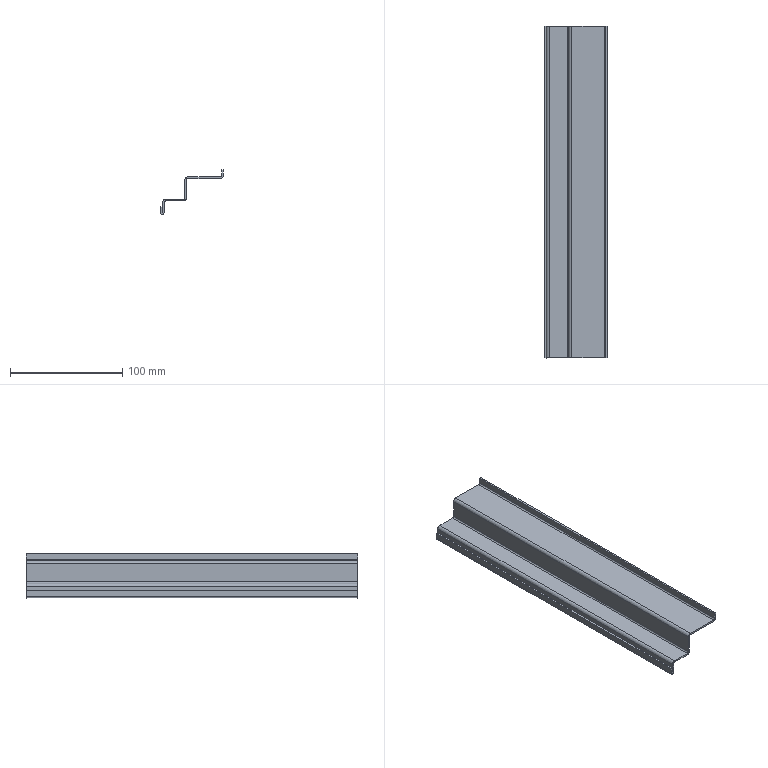Component | SolidWorks | SmallDoorFrameOne100-1 | 1 solid | 46 faces | box 56.1 x 296 x 40 mm | volume 42653 mm3 | plane 36 | cylinder 10 | commonest cylinder face diameters 5.4 x4 2.4 x4 3.1 x1 0.1 x1
STEP:
#1=COLOUR_RGB('',0.7922,0.8196,0.9333);
#2=FILL_AREA_STYLE_COLOUR('',#1);
#3=FILL_AREA_STYLE('',(#2));
#4=SURFACE_STYLE_FILL_AREA(#3);
#5=SURFACE_SIDE_STYLE('',(#4));
#6=SURFACE_STYLE_USAGE(.BOTH.,#5);
#7=PRESENTATION_STYLE_ASSIGNMENT((#6));
#8=CARTESIAN_POINT('',(32.916,29.173,17.246));
#9=VERTEX_POINT('',#8);
#10=CARTESIAN_POINT('',(32.916,29.173,17.61));
#11=VERTEX_POINT('',#10);
#12=CARTESIAN_POINT('',(32.916,29.173,17.185));
#13=DIRECTION('',(-0.,0.,1.));
#14=VECTOR('',#13,39.37);
#15=LINE('',#12,#14);
#16=EDGE_CURVE('',#9,#11,#15,.T.);
#17=ORIENTED_EDGE('',*,*,#16,.F.);
#18=CARTESIAN_POINT('',(32.975,29.173,17.246));
#19=VERTEX_POINT('',#18);
#20=CARTESIAN_POINT('',(32.916,29.173,17.246));
#21=DIRECTION('',(1.,-0.,0.));
#22=VECTOR('',#21,39.37);
#23=LINE('',#20,#22);
#24=EDGE_CURVE('',#9,#19,#23,.T.);
#25=ORIENTED_EDGE('',*,*,#24,.T.);
#26=CARTESIAN_POINT('',(32.975,29.173,17.61));
#27=VERTEX_POINT('',#26);
#28=CARTESIAN_POINT('',(32.975,29.173,17.185));
#29=DIRECTION('',(-0.,0.,1.));
#30=VECTOR('',#29,39.37);
#31=LINE('',#28,#30);
#32=EDGE_CURVE('',#19,#27,#31,.T.);
#33=ORIENTED_EDGE('',*,*,#32,.T.);
#34=CARTESIAN_POINT('',(32.975,29.173,17.61));
#35=DIRECTION('',(-1.,0.,-0.));
#36=VECTOR('',#35,39.37);
#37=LINE('',#34,#36);
#38=EDGE_CURVE('',#27,#11,#37,.T.);
#39=ORIENTED_EDGE('',*,*,#38,.T.);
#40=EDGE_LOOP('',(#17,#25,#33,#39));
#41=FACE_OUTER_BOUND('',#40,.T.);
#42=CARTESIAN_POINT('',(33.022,29.173,17.717));
#43=DIRECTION('',(-0.,-1.,0.));
#44=DIRECTION('',(0.,-0.,-1.));
#45=AXIS2_PLACEMENT_3D('',#42,#43,#44);
#46=PLANE('',#45);
#47=ADVANCED_FACE('',(#41),#46,.T.);
#48=CARTESIAN_POINT('',(33.022,40.827,17.657));
#49=VERTEX_POINT('',#48);
#50=CARTESIAN_POINT('',(33.022,40.827,17.717));
#51=VERTEX_POINT('',#50);
#52=CARTESIAN_POINT('',(33.022,40.827,17.657));
#53=DIRECTION('',(-0.,0.,1.));
#54=VECTOR('',#53,39.37);
#55=LINE('',#52,#54);
#56=EDGE_CURVE('',#49,#51,#55,.T.);
#57=ORIENTED_EDGE('',*,*,#56,.F.);
#58=CARTESIAN_POINT('',(32.975,40.827,17.61));
#59=VERTEX_POINT('',#58);
#60=CARTESIAN_POINT('',(33.022,40.827,17.61));
#61=DIRECTION('',(0.,1.,-0.));
#62=DIRECTION('',(0.,0.,-1.));
#63=AXIS2_PLACEMENT_3D('',#60,#61,#62);
#64=CIRCLE('',#63,0.04724);
#65=EDGE_CURVE('',#59,#49,#64,.T.);
#66=ORIENTED_EDGE('',*,*,#65,.F.);
#67=CARTESIAN_POINT('',(32.916,40.827,17.61));
#68=VERTEX_POINT('',#67);
#69=CARTESIAN_POINT('',(32.916,40.827,17.61));
#70=DIRECTION('',(1.,-0.,0.));
#71=VECTOR('',#70,39.37);
#72=LINE('',#69,#71);
#73=EDGE_CURVE('',#68,#59,#72,.T.);
#74=ORIENTED_EDGE('',*,*,#73,.F.);
#75=CARTESIAN_POINT('',(33.022,40.827,17.61));
#76=DIRECTION('',(0.,1.,-0.));
#77=DIRECTION('',(0.,0.,1.));
#78=AXIS2_PLACEMENT_3D('',#75,#76,#77);
#79=CIRCLE('',#78,0.1063);
#80=EDGE_CURVE('',#68,#51,#79,.T.);
#81=ORIENTED_EDGE('',*,*,#80,.T.);
#82=EDGE_LOOP('',(#57,#66,#74,#81));
#83=FACE_OUTER_BOUND('',#82,.T.);
#84=CARTESIAN_POINT('',(33.022,40.827,17.657));
#85=DIRECTION('',(0.,1.,-0.));
#86=DIRECTION('',(-0.,0.,1.));
#87=AXIS2_PLACEMENT_3D('',#84,#85,#86);
#88=PLANE('',#87);
#89=ADVANCED_FACE('',(#83),#88,.T.);
#90=CARTESIAN_POINT('',(33.656,40.827,17.657));
#91=VERTEX_POINT('',#90);
#92=CARTESIAN_POINT('',(32.975,40.827,17.657));
#93=DIRECTION('',(1.,-0.,0.));
#94=VECTOR('',#93,39.37);
#95=LINE('',#92,#94);
#96=EDGE_CURVE('',#49,#91,#95,.T.);
#97=ORIENTED_EDGE('',*,*,#96,.F.);
#98=ORIENTED_EDGE('',*,*,#56,.T.);
#99=CARTESIAN_POINT('',(33.656,40.827,17.717));
#100=VERTEX_POINT('',#99);
#101=CARTESIAN_POINT('',(32.975,40.827,17.717));
#102=DIRECTION('',(1.,-0.,0.));
#103=VECTOR('',#102,39.37);
#104=LINE('',#101,#103);
#105=EDGE_CURVE('',#51,#100,#104,.T.);
#106=ORIENTED_EDGE('',*,*,#105,.T.);
#107=CARTESIAN_POINT('',(33.656,40.827,17.717));
#108=DIRECTION('',(0.,-0.,-1.));
#109=VECTOR('',#108,39.37);
#110=LINE('',#107,#109);
#111=EDGE_CURVE('',#100,#91,#110,.T.);
#112=ORIENTED_EDGE('',*,*,#111,.T.);
#113=EDGE_LOOP('',(#97,#98,#106,#112));
#114=FACE_OUTER_BOUND('',#113,.T.);
#115=CARTESIAN_POINT('',(32.916,40.827,17.61));
#116=DIRECTION('',(0.,1.,-0.));
#117=DIRECTION('',(-0.,0.,1.));
#118=AXIS2_PLACEMENT_3D('',#115,#116,#117);
#119=PLANE('',#118);
#120=ADVANCED_FACE('',(#114),#119,.T.);
#121=ORIENTED_EDGE('',*,*,#38,.F.);
#122=CARTESIAN_POINT('',(33.022,29.173,17.657));
#123=VERTEX_POINT('',#122);
#124=CARTESIAN_POINT('',(33.022,29.173,17.61));
#125=DIRECTION('',(0.,1.,-0.));
#126=DIRECTION('',(0.,0.,-1.));
#127=AXIS2_PLACEMENT_3D('',#124,#125,#126);
#128=CIRCLE('',#127,0.04724);
#129=EDGE_CURVE('',#27,#123,#128,.T.);
#130=ORIENTED_EDGE('',*,*,#129,.T.);
#131=CARTESIAN_POINT('',(33.022,29.173,17.717));
#132=VERTEX_POINT('',#131);
#133=CARTESIAN_POINT('',(33.022,29.173,17.717));
#134=DIRECTION('',(0.,-0.,-1.));
#135=VECTOR('',#134,39.37);
#136=LINE('',#133,#135);
#137=EDGE_CURVE('',#132,#123,#136,.T.);
#138=ORIENTED_EDGE('',*,*,#137,.F.);
#139=CARTESIAN_POINT('',(33.022,29.173,17.61));
#140=DIRECTION('',(0.,1.,-0.));
#141=DIRECTION('',(0.,0.,1.));
#142=AXIS2_PLACEMENT_3D('',#139,#140,#141);
#143=CIRCLE('',#142,0.1063);
#144=EDGE_CURVE('',#11,#132,#143,.T.);
#145=ORIENTED_EDGE('',*,*,#144,.F.);
#146=EDGE_LOOP('',(#121,#130,#138,#145));
#147=FACE_OUTER_BOUND('',#146,.T.);
#148=CARTESIAN_POINT('',(32.975,29.173,17.61));
#149=DIRECTION('',(-0.,-1.,0.));
#150=DIRECTION('',(0.,-0.,-1.));
#151=AXIS2_PLACEMENT_3D('',#148,#149,#150);
#152=PLANE('',#151);
#153=ADVANCED_FACE('',(#147),#152,.T.);
#154=CARTESIAN_POINT('',(33.762,40.827,17.764));
#155=VERTEX_POINT('',#154);
#156=CARTESIAN_POINT('',(33.703,40.827,17.764));
#157=VERTEX_POINT('',#156);
#158=CARTESIAN_POINT('',(33.762,40.827,17.764));
#159=DIRECTION('',(-1.,0.,-0.));
#160=VECTOR('',#159,39.37);
#161=LINE('',#158,#160);
#162=EDGE_CURVE('',#155,#157,#161,.T.);
#163=ORIENTED_EDGE('',*,*,#162,.F.);
#164=CARTESIAN_POINT('',(33.656,40.827,17.764));
#165=DIRECTION('',(-0.,-1.,0.));
#166=DIRECTION('',(0.,0.,1.));
#167=AXIS2_PLACEMENT_3D('',#164,#165,#166);
#168=CIRCLE('',#167,0.1063);
#169=EDGE_CURVE('',#91,#155,#168,.T.);
#170=ORIENTED_EDGE('',*,*,#169,.F.);
#171=ORIENTED_EDGE('',*,*,#111,.F.);
#172=CARTESIAN_POINT('',(33.656,40.827,17.764));
#173=DIRECTION('',(-0.,-1.,0.));
#174=DIRECTION('',(0.,0.,1.));
#175=AXIS2_PLACEMENT_3D('',#172,#173,#174);
#176=CIRCLE('',#175,0.04724);
#177=EDGE_CURVE('',#100,#157,#176,.T.);
#178=ORIENTED_EDGE('',*,*,#177,.T.);
#179=EDGE_LOOP('',(#163,#170,#171,#178));
#180=FACE_OUTER_BOUND('',#179,.T.);
#181=CARTESIAN_POINT('',(33.762,40.827,17.764));
#182=DIRECTION('',(0.,1.,-0.));
#183=DIRECTION('',(-0.,0.,1.));
#184=AXIS2_PLACEMENT_3D('',#181,#182,#183);
#185=PLANE('',#184);
#186=ADVANCED_FACE('',(#180),#185,.T.);
#187=CARTESIAN_POINT('',(33.762,40.827,18.398));
#188=VERTEX_POINT('',#187);
#189=CARTESIAN_POINT('',(33.762,40.827,17.657));
#190=DIRECTION('',(-0.,0.,1.));
#191=VECTOR('',#190,39.37);
#192=LINE('',#189,#191);
#193=EDGE_CURVE('',#155,#188,#192,.T.);
#194=ORIENTED_EDGE('',*,*,#193,.F.);
#195=ORIENTED_EDGE('',*,*,#162,.T.);
#196=CARTESIAN_POINT('',(33.703,40.827,18.398));
#197=VERTEX_POINT('',#196);
#198=CARTESIAN_POINT('',(33.703,40.827,17.657));
#199=DIRECTION('',(-0.,0.,1.));
#200=VECTOR('',#199,39.37);
#201=LINE('',#198,#200);
#202=EDGE_CURVE('',#157,#197,#201,.T.);
#203=ORIENTED_EDGE('',*,*,#202,.T.);
#204=CARTESIAN_POINT('',(33.703,40.827,18.398));
#205=DIRECTION('',(1.,-0.,0.));
#206=VECTOR('',#205,39.37);
#207=LINE('',#204,#206);
#208=EDGE_CURVE('',#197,#188,#207,.T.);
#209=ORIENTED_EDGE('',*,*,#208,.T.);
#210=EDGE_LOOP('',(#194,#195,#203,#209));
#211=FACE_OUTER_BOUND('',#210,.T.);
#212=CARTESIAN_POINT('',(33.656,40.827,17.717));
#213=DIRECTION('',(0.,1.,-0.));
#214=DIRECTION('',(-0.,0.,1.));
#215=AXIS2_PLACEMENT_3D('',#212,#213,#214);
#216=PLANE('',#215);
#217=ADVANCED_FACE('',(#211),#216,.T.);
#218=CARTESIAN_POINT('',(33.656,29.173,17.657));
#219=VERTEX_POINT('',#218);
#220=CARTESIAN_POINT('',(33.656,29.173,17.717));
#221=VERTEX_POINT('',#220);
#222=CARTESIAN_POINT('',(33.656,29.173,17.657));
#223=DIRECTION('',(-0.,0.,1.));
#224=VECTOR('',#223,39.37);
#225=LINE('',#222,#224);
#226=EDGE_CURVE('',#219,#221,#225,.T.);
#227=ORIENTED_EDGE('',*,*,#226,.F.);
#228=CARTESIAN_POINT('',(33.762,29.173,17.764));
#229=VERTEX_POINT('',#228);
#230=CARTESIAN_POINT('',(33.656,29.173,17.764));
#231=DIRECTION('',(-0.,-1.,0.));
#232=DIRECTION('',(0.,0.,1.));
#233=AXIS2_PLACEMENT_3D('',#230,#231,#232);
#234=CIRCLE('',#233,0.1063);
#235=EDGE_CURVE('',#219,#229,#234,.T.);
#236=ORIENTED_EDGE('',*,*,#235,.T.);
#237=CARTESIAN_POINT('',(33.703,29.173,17.764));
#238=VERTEX_POINT('',#237);
#239=CARTESIAN_POINT('',(33.703,29.173,17.764));
#240=DIRECTION('',(1.,-0.,0.));
#241=VECTOR('',#240,39.37);
#242=LINE('',#239,#241);
#243=EDGE_CURVE('',#238,#229,#242,.T.);
#244=ORIENTED_EDGE('',*,*,#243,.F.);
#245=CARTESIAN_POINT('',(33.656,29.173,17.764));
#246=DIRECTION('',(-0.,-1.,0.));
#247=DIRECTION('',(0.,0.,1.));
#248=AXIS2_PLACEMENT_3D('',#245,#246,#247);
#249=CIRCLE('',#248,0.04724);
#250=EDGE_CURVE('',#221,#238,#249,.T.);
#251=ORIENTED_EDGE('',*,*,#250,.F.);
#252=EDGE_LOOP('',(#227,#236,#244,#251));
#253=FACE_OUTER_BOUND('',#252,.T.);
#254=CARTESIAN_POINT('',(33.656,29.173,17.657));
#255=DIRECTION('',(-0.,-1.,0.));
#256=DIRECTION('',(0.,-0.,-1.));
#257=AXIS2_PLACEMENT_3D('',#254,#255,#256);
#258=PLANE('',#257);
#259=ADVANCED_FACE('',(#253),#258,.T.);
#260=CARTESIAN_POINT('',(32.975,29.173,17.657));
#261=DIRECTION('',(1.,-0.,0.));
#262=VECTOR('',#261,39.37);
#263=LINE('',#260,#262);
#264=EDGE_CURVE('',#123,#219,#263,.T.);
#265=ORIENTED_EDGE('',*,*,#264,.T.);
#266=ORIENTED_EDGE('',*,*,#226,.T.);
#267=CARTESIAN_POINT('',(32.975,29.173,17.717));
#268=DIRECTION('',(1.,-0.,0.));
#269=VECTOR('',#268,39.37);
#270=LINE('',#267,#269);
#271=EDGE_CURVE('',#132,#221,#270,.T.);
#272=ORIENTED_EDGE('',*,*,#271,.F.);
#273=ORIENTED_EDGE('',*,*,#137,.T.);
#274=EDGE_LOOP('',(#265,#266,#272,#273));
#275=FACE_OUTER_BOUND('',#274,.T.);
#276=CARTESIAN_POINT('',(33.703,29.173,17.764));
#277=DIRECTION('',(-0.,-1.,0.));
#278=DIRECTION('',(0.,-0.,-1.));
#279=AXIS2_PLACEMENT_3D('',#276,#277,#278);
#280=PLANE('',#279);
#281=ADVANCED_FACE('',(#275),#280,.T.);
#282=CARTESIAN_POINT('',(33.809,40.827,18.445));
#283=VERTEX_POINT('',#282);
#284=CARTESIAN_POINT('',(33.809,40.827,18.504));
#285=VERTEX_POINT('',#284);
#286=CARTESIAN_POINT('',(33.809,40.827,18.445));
#287=DIRECTION('',(-0.,0.,1.));
#288=VECTOR('',#287,39.37);
#289=LINE('',#286,#288);
#290=EDGE_CURVE('',#283,#285,#289,.T.);
#291=ORIENTED_EDGE('',*,*,#290,.F.);
#292=CARTESIAN_POINT('',(33.809,40.827,18.398));
#293=DIRECTION('',(0.,1.,-0.));
#294=DIRECTION('',(0.,0.,-1.));
#295=AXIS2_PLACEMENT_3D('',#292,#293,#294);
#296=CIRCLE('',#295,0.04724);
#297=EDGE_CURVE('',#188,#283,#296,.T.);
#298=ORIENTED_EDGE('',*,*,#297,.F.);
#299=ORIENTED_EDGE('',*,*,#208,.F.);
#300=CARTESIAN_POINT('',(33.809,40.827,18.398));
#301=DIRECTION('',(0.,1.,-0.));
#302=DIRECTION('',(0.,0.,1.));
#303=AXIS2_PLACEMENT_3D('',#300,#301,#302);
#304=CIRCLE('',#303,0.1063);
#305=EDGE_CURVE('',#197,#285,#304,.T.);
#306=ORIENTED_EDGE('',*,*,#305,.T.);
#307=EDGE_LOOP('',(#291,#298,#299,#306));
#308=FACE_OUTER_BOUND('',#307,.T.);
#309=CARTESIAN_POINT('',(33.809,40.827,18.445));
#310=DIRECTION('',(0.,1.,-0.));
#311=DIRECTION('',(-0.,0.,1.));
#312=AXIS2_PLACEMENT_3D('',#309,#310,#311);
#313=PLANE('',#312);
#314=ADVANCED_FACE('',(#308),#313,.T.);
#315=CARTESIAN_POINT('',(34.955,40.827,18.445));
#316=VERTEX_POINT('',#315);
#317=CARTESIAN_POINT('',(33.762,40.827,18.445));
#318=DIRECTION('',(1.,-0.,0.));
#319=VECTOR('',#318,39.37);
#320=LINE('',#317,#319);
#321=EDGE_CURVE('',#283,#316,#320,.T.);
#322=ORIENTED_EDGE('',*,*,#321,.F.);
#323=ORIENTED_EDGE('',*,*,#290,.T.);
#324=CARTESIAN_POINT('',(34.955,40.827,18.504));
#325=VERTEX_POINT('',#324);
#326=CARTESIAN_POINT('',(33.762,40.827,18.504));
#327=DIRECTION('',(1.,-0.,0.));
#328=VECTOR('',#327,39.37);
#329=LINE('',#326,#328);
#330=EDGE_CURVE('',#285,#325,#329,.T.);
#331=ORIENTED_EDGE('',*,*,#330,.T.);
#332=CARTESIAN_POINT('',(34.955,40.827,18.504));
#333=DIRECTION('',(0.,-0.,-1.));
#334=VECTOR('',#333,39.37);
#335=LINE('',#332,#334);
#336=EDGE_CURVE('',#325,#316,#335,.T.);
#337=ORIENTED_EDGE('',*,*,#336,.T.);
#338=EDGE_LOOP('',(#322,#323,#331,#337));
#339=FACE_OUTER_BOUND('',#338,.T.);
#340=CARTESIAN_POINT('',(33.703,40.827,18.398));
#341=DIRECTION('',(0.,1.,-0.));
#342=DIRECTION('',(-0.,0.,1.));
#343=AXIS2_PLACEMENT_3D('',#340,#341,#342);
#344=PLANE('',#343);
#345=ADVANCED_FACE('',(#339),#344,.T.);
#346=CARTESIAN_POINT('',(33.762,29.173,18.398));
#347=VERTEX_POINT('',#346);
#348=CARTESIAN_POINT('',(33.703,29.173,18.398));
#349=VERTEX_POINT('',#348);
#350=CARTESIAN_POINT('',(33.762,29.173,18.398));
#351=DIRECTION('',(-1.,0.,-0.));
#352=VECTOR('',#351,39.37);
#353=LINE('',#350,#352);
#354=EDGE_CURVE('',#347,#349,#353,.T.);
#355=ORIENTED_EDGE('',*,*,#354,.F.);
#356=CARTESIAN_POINT('',(33.809,29.173,18.445));
#357=VERTEX_POINT('',#356);
#358=CARTESIAN_POINT('',(33.809,29.173,18.398));
#359=DIRECTION('',(0.,1.,-0.));
#360=DIRECTION('',(0.,0.,-1.));
#361=AXIS2_PLACEMENT_3D('',#358,#359,#360);
#362=CIRCLE('',#361,0.04724);
#363=EDGE_CURVE('',#347,#357,#362,.T.);
#364=ORIENTED_EDGE('',*,*,#363,.T.);
#365=CARTESIAN_POINT('',(33.809,29.173,18.504));
#366=VERTEX_POINT('',#365);
#367=CARTESIAN_POINT('',(33.809,29.173,18.504));
#368=DIRECTION('',(0.,-0.,-1.));
#369=VECTOR('',#368,39.37);
#370=LINE('',#367,#369);
#371=EDGE_CURVE('',#366,#357,#370,.T.);
#372=ORIENTED_EDGE('',*,*,#371,.F.);
#373=CARTESIAN_POINT('',(33.809,29.173,18.398));
#374=DIRECTION('',(0.,1.,-0.));
#375=DIRECTION('',(0.,0.,1.));
#376=AXIS2_PLACEMENT_3D('',#373,#374,#375);
#377=CIRCLE('',#376,0.1063);
#378=EDGE_CURVE('',#349,#366,#377,.T.);
#379=ORIENTED_EDGE('',*,*,#378,.F.);
#380=EDGE_LOOP('',(#355,#364,#372,#379));
#381=FACE_OUTER_BOUND('',#380,.T.);
#382=CARTESIAN_POINT('',(33.762,29.173,18.398));
#383=DIRECTION('',(-0.,-1.,0.));
#384=DIRECTION('',(0.,-0.,-1.));
#385=AXIS2_PLACEMENT_3D('',#382,#383,#384);
#386=PLANE('',#385);
#387=ADVANCED_FACE('',(#381),#386,.T.);
#388=CARTESIAN_POINT('',(33.762,29.173,17.657));
#389=DIRECTION('',(-0.,0.,1.));
#390=VECTOR('',#389,39.37);
#391=LINE('',#388,#390);
#392=EDGE_CURVE('',#229,#347,#391,.T.);
#393=ORIENTED_EDGE('',*,*,#392,.T.);
#394=ORIENTED_EDGE('',*,*,#354,.T.);
#395=CARTESIAN_POINT('',(33.703,29.173,17.657));
#396=DIRECTION('',(-0.,0.,1.));
#397=VECTOR('',#396,39.37);
#398=LINE('',#395,#397);
#399=EDGE_CURVE('',#238,#349,#398,.T.);
#400=ORIENTED_EDGE('',*,*,#399,.F.);
#401=ORIENTED_EDGE('',*,*,#243,.T.);
#402=EDGE_LOOP('',(#393,#394,#400,#401));
#403=FACE_OUTER_BOUND('',#402,.T.);
#404=CARTESIAN_POINT('',(33.809,29.173,18.504));
#405=DIRECTION('',(-0.,-1.,0.));
#406=DIRECTION('',(0.,-0.,-1.));
#407=AXIS2_PLACEMENT_3D('',#404,#405,#406);
#408=PLANE('',#407);
#409=ADVANCED_FACE('',(#403),#408,.T.);
#410=CARTESIAN_POINT('',(35.061,40.827,18.551));
#411=VERTEX_POINT('',#410);
#412=CARTESIAN_POINT('',(35.002,40.827,18.551));
#413=VERTEX_POINT('',#412);
#414=CARTESIAN_POINT('',(35.061,40.827,18.551));
#415=DIRECTION('',(-1.,0.,-0.));
#416=VECTOR('',#415,39.37);
#417=LINE('',#414,#416);
#418=EDGE_CURVE('',#411,#413,#417,.T.);
#419=ORIENTED_EDGE('',*,*,#418,.F.);
#420=CARTESIAN_POINT('',(34.955,40.827,18.551));
#421=DIRECTION('',(-0.,-1.,0.));
#422=DIRECTION('',(0.,0.,1.));
#423=AXIS2_PLACEMENT_3D('',#420,#421,#422);
#424=CIRCLE('',#423,0.1063);
#425=EDGE_CURVE('',#316,#411,#424,.T.);
#426=ORIENTED_EDGE('',*,*,#425,.F.);
#427=ORIENTED_EDGE('',*,*,#336,.F.);
#428=CARTESIAN_POINT('',(34.955,40.827,18.551));
#429=DIRECTION('',(-0.,-1.,0.));
#430=DIRECTION('',(0.,0.,1.));
#431=AXIS2_PLACEMENT_3D('',#428,#429,#430);
#432=CIRCLE('',#431,0.04724);
#433=EDGE_CURVE('',#325,#413,#432,.T.);
#434=ORIENTED_EDGE('',*,*,#433,.T.);
#435=EDGE_LOOP('',(#419,#426,#427,#434));
#436=FACE_OUTER_BOUND('',#435,.T.);
#437=CARTESIAN_POINT('',(35.061,40.827,18.551));
#438=DIRECTION('',(0.,1.,-0.));
#439=DIRECTION('',(-0.,0.,1.));
#440=AXIS2_PLACEMENT_3D('',#437,#438,#439);
#441=PLANE('',#440);
#442=ADVANCED_FACE('',(#436),#441,.T.);
#443=CARTESIAN_POINT('',(35.061,40.827,18.76));
#444=VERTEX_POINT('',#443);
#445=CARTESIAN_POINT('',(35.061,40.827,18.445));
#446=DIRECTION('',(-0.,0.,1.));
#447=VECTOR('',#446,39.37);
#448=LINE('',#445,#447);
#449=EDGE_CURVE('',#411,#444,#448,.T.);
#450=ORIENTED_EDGE('',*,*,#449,.F.);
#451=ORIENTED_EDGE('',*,*,#418,.T.);
#452=CARTESIAN_POINT('',(35.002,40.827,18.76));
#453=VERTEX_POINT('',#452);
#454=CARTESIAN_POINT('',(35.002,40.827,18.445));
#455=DIRECTION('',(-0.,0.,1.));
#456=VECTOR('',#455,39.37);
#457=LINE('',#454,#456);
#458=EDGE_CURVE('',#413,#453,#457,.T.);
#459=ORIENTED_EDGE('',*,*,#458,.T.);
#460=CARTESIAN_POINT('',(35.061,40.827,18.76));
#461=DIRECTION('',(-1.,0.,-0.));
#462=VECTOR('',#461,39.37);
#463=LINE('',#460,#462);
#464=EDGE_CURVE('',#444,#453,#463,.T.);
#465=ORIENTED_EDGE('',*,*,#464,.F.);
#466=EDGE_LOOP('',(#450,#451,#459,#465));
#467=FACE_OUTER_BOUND('',#466,.T.);
#468=CARTESIAN_POINT('',(34.955,40.827,18.504));
#469=DIRECTION('',(0.,1.,-0.));
#470=DIRECTION('',(-0.,0.,1.));
#471=AXIS2_PLACEMENT_3D('',#468,#469,#470);
#472=PLANE('',#471);
#473=ADVANCED_FACE('',(#467),#472,.T.);
#474=CARTESIAN_POINT('',(34.955,29.173,18.445));
#475=VERTEX_POINT('',#474);
#476=CARTESIAN_POINT('',(34.955,29.173,18.504));
#477=VERTEX_POINT('',#476);
#478=CARTESIAN_POINT('',(34.955,29.173,18.445));
#479=DIRECTION('',(-0.,0.,1.));
#480=VECTOR('',#479,39.37);
#481=LINE('',#478,#480);
#482=EDGE_CURVE('',#475,#477,#481,.T.);
#483=ORIENTED_EDGE('',*,*,#482,.F.);
#484=CARTESIAN_POINT('',(35.061,29.173,18.551));
#485=VERTEX_POINT('',#484);
#486=CARTESIAN_POINT('',(34.955,29.173,18.551));
#487=DIRECTION('',(-0.,-1.,0.));
#488=DIRECTION('',(0.,0.,1.));
#489=AXIS2_PLACEMENT_3D('',#486,#487,#488);
#490=CIRCLE('',#489,0.1063);
#491=EDGE_CURVE('',#475,#485,#490,.T.);
#492=ORIENTED_EDGE('',*,*,#491,.T.);
#493=CARTESIAN_POINT('',(35.002,29.173,18.551));
#494=VERTEX_POINT('',#493);
#495=CARTESIAN_POINT('',(35.002,29.173,18.551));
#496=DIRECTION('',(1.,-0.,0.));
#497=VECTOR('',#496,39.37);
#498=LINE('',#495,#497);
#499=EDGE_CURVE('',#494,#485,#498,.T.);
#500=ORIENTED_EDGE('',*,*,#499,.F.);
#501=CARTESIAN_POINT('',(34.955,29.173,18.551));
#502=DIRECTION('',(-0.,-1.,0.));
#503=DIRECTION('',(0.,0.,1.));
#504=AXIS2_PLACEMENT_3D('',#501,#502,#503);
#505=CIRCLE('',#504,0.04724);
#506=EDGE_CURVE('',#477,#494,#505,.T.);
#507=ORIENTED_EDGE('',*,*,#506,.F.);
#508=EDGE_LOOP('',(#483,#492,#500,#507));
#509=FACE_OUTER_BOUND('',#508,.T.);
#510=CARTESIAN_POINT('',(34.955,29.173,18.445));
#511=DIRECTION('',(-0.,-1.,0.));
#512=DIRECTION('',(0.,-0.,-1.));
#513=AXIS2_PLACEMENT_3D('',#510,#511,#512);
#514=PLANE('',#513);
#515=ADVANCED_FACE('',(#509),#514,.T.);
#516=CARTESIAN_POINT('',(33.762,29.173,18.445));
#517=DIRECTION('',(1.,-0.,0.));
#518=VECTOR('',#517,39.37);
#519=LINE('',#516,#518);
#520=EDGE_CURVE('',#357,#475,#519,.T.);
#521=ORIENTED_EDGE('',*,*,#520,.T.);
#522=ORIENTED_EDGE('',*,*,#482,.T.);
#523=CARTESIAN_POINT('',(33.762,29.173,18.504));
#524=DIRECTION('',(1.,-0.,0.));
#525=VECTOR('',#524,39.37);
#526=LINE('',#523,#525);
#527=EDGE_CURVE('',#366,#477,#526,.T.);
#528=ORIENTED_EDGE('',*,*,#527,.F.);
#529=ORIENTED_EDGE('',*,*,#371,.T.);
#530=EDGE_LOOP('',(#521,#522,#528,#529));
#531=FACE_OUTER_BOUND('',#530,.T.);
#532=CARTESIAN_POINT('',(35.002,29.173,18.551));
#533=DIRECTION('',(-0.,-1.,0.));
#534=DIRECTION('',(0.,-0.,-1.));
#535=AXIS2_PLACEMENT_3D('',#532,#533,#534);
#536=PLANE('',#535);
#537=ADVANCED_FACE('',(#531),#536,.T.);
#538=CARTESIAN_POINT('',(35.002,29.173,18.76));
#539=VERTEX_POINT('',#538);
#540=CARTESIAN_POINT('',(35.002,29.173,18.445));
#541=DIRECTION('',(-0.,0.,1.));
#542=VECTOR('',#541,39.37);
#543=LINE('',#540,#542);
#544=EDGE_CURVE('',#494,#539,#543,.T.);
#545=ORIENTED_EDGE('',*,*,#544,.T.);
#546=CARTESIAN_POINT('',(35.002,40.827,18.76));
#547=DIRECTION('',(-0.,-1.,0.));
#548=VECTOR('',#547,39.37);
#549=LINE('',#546,#548);
#550=EDGE_CURVE('',#453,#539,#549,.T.);
#551=ORIENTED_EDGE('',*,*,#550,.F.);
#552=ORIENTED_EDGE('',*,*,#458,.F.);
#553=CARTESIAN_POINT('',(35.002,40.827,18.551));
#554=DIRECTION('',(-0.,-1.,0.));
#555=VECTOR('',#554,39.37);
#556=LINE('',#553,#555);
#557=EDGE_CURVE('',#413,#494,#556,.T.);
#558=ORIENTED_EDGE('',*,*,#557,.T.);
#559=EDGE_LOOP('',(#545,#551,#552,#558));
#560=FACE_OUTER_BOUND('',#559,.T.);
#561=CARTESIAN_POINT('',(35.002,40.827,18.445));
#562=DIRECTION('',(1.,-0.,0.));
#563=DIRECTION('',(0.,1.,-0.));
#564=AXIS2_PLACEMENT_3D('',#561,#562,#563);
#565=PLANE('',#564);
#566=ADVANCED_FACE('',(#560),#565,.F.);
#567=CARTESIAN_POINT('',(35.061,29.173,18.76));
#568=VERTEX_POINT('',#567);
#569=CARTESIAN_POINT('',(35.061,29.173,18.76));
#570=DIRECTION('',(-1.,0.,-0.));
#571=VECTOR('',#570,39.37);
#572=LINE('',#569,#571);
#573=EDGE_CURVE('',#568,#539,#572,.T.);
#574=ORIENTED_EDGE('',*,*,#573,.F.);
#575=CARTESIAN_POINT('',(35.061,40.827,18.76));
#576=DIRECTION('',(-0.,-1.,0.));
#577=VECTOR('',#576,39.37);
#578=LINE('',#575,#577);
#579=EDGE_CURVE('',#444,#568,#578,.T.);
#580=ORIENTED_EDGE('',*,*,#579,.F.);
#581=ORIENTED_EDGE('',*,*,#464,.T.);
#582=ORIENTED_EDGE('',*,*,#550,.T.);
#583=EDGE_LOOP('',(#574,#580,#581,#582));
#584=FACE_OUTER_BOUND('',#583,.T.);
#585=CARTESIAN_POINT('',(35.061,40.827,18.76));
#586=DIRECTION('',(-0.,0.,1.));
#587=DIRECTION('',(-0.,-1.,0.));
#588=AXIS2_PLACEMENT_3D('',#585,#586,#587);
#589=PLANE('',#588);
#590=ADVANCED_FACE('',(#584),#589,.T.);
#591=CARTESIAN_POINT('',(35.061,29.173,18.445));
#592=DIRECTION('',(-0.,0.,1.));
#593=VECTOR('',#592,39.37);
#594=LINE('',#591,#593);
#595=EDGE_CURVE('',#485,#568,#594,.T.);
#596=ORIENTED_EDGE('',*,*,#595,.F.);
#597=CARTESIAN_POINT('',(35.061,40.827,18.551));
#598=DIRECTION('',(-0.,-1.,0.));
#599=VECTOR('',#598,39.37);
#600=LINE('',#597,#599);
#601=EDGE_CURVE('',#411,#485,#600,.T.);
#602=ORIENTED_EDGE('',*,*,#601,.F.);
#603=ORIENTED_EDGE('',*,*,#449,.T.);
#604=ORIENTED_EDGE('',*,*,#579,.T.);
#605=EDGE_LOOP('',(#596,#602,#603,#604));
#606=FACE_OUTER_BOUND('',#605,.T.);
#607=CARTESIAN_POINT('',(35.061,40.827,18.445));
#608=DIRECTION('',(1.,-0.,0.));
#609=DIRECTION('',(0.,1.,-0.));
#610=AXIS2_PLACEMENT_3D('',#607,#608,#609);
#611=PLANE('',#610);
#612=ADVANCED_FACE('',(#606),#611,.T.);
#613=ORIENTED_EDGE('',*,*,#491,.F.);
#614=CARTESIAN_POINT('',(34.955,40.827,18.445));
#615=DIRECTION('',(-0.,-1.,0.));
#616=VECTOR('',#615,39.37);
#617=LINE('',#614,#616);
#618=EDGE_CURVE('',#316,#475,#617,.T.);
#619=ORIENTED_EDGE('',*,*,#618,.F.);
#620=ORIENTED_EDGE('',*,*,#425,.T.);
#621=ORIENTED_EDGE('',*,*,#601,.T.);
#622=EDGE_LOOP('',(#613,#619,#620,#621));
#623=FACE_OUTER_BOUND('',#622,.T.);
#624=CARTESIAN_POINT('',(34.955,40.827,18.551));
#625=DIRECTION('',(-0.,-1.,0.));
#626=DIRECTION('',(0.,0.,-1.));
#627=AXIS2_PLACEMENT_3D('',#624,#625,#626);
#628=CYLINDRICAL_SURFACE('',#627,0.1063);
#629=ADVANCED_FACE('',(#623),#628,.T.);
#630=ORIENTED_EDGE('',*,*,#520,.F.);
#631=CARTESIAN_POINT('',(33.809,40.827,18.445));
#632=DIRECTION('',(-0.,-1.,0.));
#633=VECTOR('',#632,39.37);
#634=LINE('',#631,#633);
#635=EDGE_CURVE('',#283,#357,#634,.T.);
#636=ORIENTED_EDGE('',*,*,#635,.F.);
#637=ORIENTED_EDGE('',*,*,#321,.T.);
#638=ORIENTED_EDGE('',*,*,#618,.T.);
#639=EDGE_LOOP('',(#630,#636,#637,#638));
#640=FACE_OUTER_BOUND('',#639,.T.);
#641=CARTESIAN_POINT('',(33.762,40.827,18.445));
#642=DIRECTION('',(0.,-0.,-1.));
#643=DIRECTION('',(0.,1.,-0.));
#644=AXIS2_PLACEMENT_3D('',#641,#642,#643);
#645=PLANE('',#644);
#646=ADVANCED_FACE('',(#640),#645,.T.);
#647=ORIENTED_EDGE('',*,*,#363,.F.);
#648=CARTESIAN_POINT('',(33.762,40.827,18.398));
#649=DIRECTION('',(-0.,-1.,0.));
#650=VECTOR('',#649,39.37);
#651=LINE('',#648,#650);
#652=EDGE_CURVE('',#188,#347,#651,.T.);
#653=ORIENTED_EDGE('',*,*,#652,.F.);
#654=ORIENTED_EDGE('',*,*,#297,.T.);
#655=ORIENTED_EDGE('',*,*,#635,.T.);
#656=EDGE_LOOP('',(#647,#653,#654,#655));
#657=FACE_OUTER_BOUND('',#656,.T.);
#658=CARTESIAN_POINT('',(33.809,40.827,18.398));
#659=DIRECTION('',(-0.,-1.,0.));
#660=DIRECTION('',(0.,0.,-1.));
#661=AXIS2_PLACEMENT_3D('',#658,#659,#660);
#662=CYLINDRICAL_SURFACE('',#661,0.04724);
#663=ADVANCED_FACE('',(#657),#662,.F.);
#664=ORIENTED_EDGE('',*,*,#392,.F.);
#665=CARTESIAN_POINT('',(33.762,40.827,17.764));
#666=DIRECTION('',(-0.,-1.,0.));
#667=VECTOR('',#666,39.37);
#668=LINE('',#665,#667);
#669=EDGE_CURVE('',#155,#229,#668,.T.);
#670=ORIENTED_EDGE('',*,*,#669,.F.);
#671=ORIENTED_EDGE('',*,*,#193,.T.);
#672=ORIENTED_EDGE('',*,*,#652,.T.);
#673=EDGE_LOOP('',(#664,#670,#671,#672));
#674=FACE_OUTER_BOUND('',#673,.T.);
#675=CARTESIAN_POINT('',(33.762,40.827,17.657));
#676=DIRECTION('',(1.,-0.,0.));
#677=DIRECTION('',(0.,1.,-0.));
#678=AXIS2_PLACEMENT_3D('',#675,#676,#677);
#679=PLANE('',#678);
#680=ADVANCED_FACE('',(#674),#679,.T.);
#681=ORIENTED_EDGE('',*,*,#235,.F.);
#682=CARTESIAN_POINT('',(33.656,40.827,17.657));
#683=DIRECTION('',(-0.,-1.,0.));
#684=VECTOR('',#683,39.37);
#685=LINE('',#682,#684);
#686=EDGE_CURVE('',#91,#219,#685,.T.);
#687=ORIENTED_EDGE('',*,*,#686,.F.);
#688=ORIENTED_EDGE('',*,*,#169,.T.);
#689=ORIENTED_EDGE('',*,*,#669,.T.);
#690=EDGE_LOOP('',(#681,#687,#688,#689));
#691=FACE_OUTER_BOUND('',#690,.T.);
#692=CARTESIAN_POINT('',(33.656,40.827,17.764));
#693=DIRECTION('',(-0.,-1.,0.));
#694=DIRECTION('',(0.,0.,-1.));
#695=AXIS2_PLACEMENT_3D('',#692,#693,#694);
#696=CYLINDRICAL_SURFACE('',#695,0.1063);
#697=ADVANCED_FACE('',(#691),#696,.T.);
#698=ORIENTED_EDGE('',*,*,#264,.F.);
#699=CARTESIAN_POINT('',(33.022,40.827,17.657));
#700=DIRECTION('',(-0.,-1.,0.));
#701=VECTOR('',#700,39.37);
#702=LINE('',#699,#701);
#703=EDGE_CURVE('',#49,#123,#702,.T.);
#704=ORIENTED_EDGE('',*,*,#703,.F.);
#705=ORIENTED_EDGE('',*,*,#96,.T.);
#706=ORIENTED_EDGE('',*,*,#686,.T.);
#707=EDGE_LOOP('',(#698,#704,#705,#706));
#708=FACE_OUTER_BOUND('',#707,.T.);
#709=CARTESIAN_POINT('',(32.975,40.827,17.657));
#710=DIRECTION('',(0.,-0.,-1.));
#711=DIRECTION('',(0.,1.,-0.));
#712=AXIS2_PLACEMENT_3D('',#709,#710,#711);
#713=PLANE('',#712);
#714=ADVANCED_FACE('',(#708),#713,.T.);
#715=ORIENTED_EDGE('',*,*,#129,.F.);
#716=CARTESIAN_POINT('',(32.975,40.827,17.61));
#717=DIRECTION('',(-0.,-1.,0.));
#718=VECTOR('',#717,39.37);
#719=LINE('',#716,#718);
#720=EDGE_CURVE('',#59,#27,#719,.T.);
#721=ORIENTED_EDGE('',*,*,#720,.F.);
#722=ORIENTED_EDGE('',*,*,#65,.T.);
#723=ORIENTED_EDGE('',*,*,#703,.T.);
#724=EDGE_LOOP('',(#715,#721,#722,#723));
#725=FACE_OUTER_BOUND('',#724,.T.);
#726=CARTESIAN_POINT('',(33.022,40.827,17.61));
#727=DIRECTION('',(-0.,-1.,0.));
#728=DIRECTION('',(0.,0.,-1.));
#729=AXIS2_PLACEMENT_3D('',#726,#727,#728);
#730=CYLINDRICAL_SURFACE('',#729,0.04724);
#731=ADVANCED_FACE('',(#725),#730,.F.);
#732=CARTESIAN_POINT('',(32.975,40.827,17.246));
#733=VERTEX_POINT('',#732);
#734=CARTESIAN_POINT('',(32.975,29.173,17.246));
#735=DIRECTION('',(0.,1.,-0.));
#736=VECTOR('',#735,39.37);
#737=LINE('',#734,#736);
#738=EDGE_CURVE('',#19,#733,#737,.T.);
#739=ORIENTED_EDGE('',*,*,#738,.T.);
#740=CARTESIAN_POINT('',(32.975,40.827,17.185));
#741=DIRECTION('',(-0.,0.,1.));
#742=VECTOR('',#741,39.37);
#743=LINE('',#740,#742);
#744=EDGE_CURVE('',#733,#59,#743,.T.);
#745=ORIENTED_EDGE('',*,*,#744,.T.);
#746=ORIENTED_EDGE('',*,*,#720,.T.);
#747=ORIENTED_EDGE('',*,*,#32,.F.);
#748=EDGE_LOOP('',(#739,#745,#746,#747));
#749=FACE_OUTER_BOUND('',#748,.T.);
#750=CARTESIAN_POINT('',(32.975,40.827,17.185));
#751=DIRECTION('',(1.,-0.,0.));
#752=DIRECTION('',(0.,1.,-0.));
#753=AXIS2_PLACEMENT_3D('',#750,#751,#752);
#754=PLANE('',#753);
#755=ADVANCED_FACE('',(#749),#754,.T.);
#756=CARTESIAN_POINT('',(32.916,40.827,17.246));
#757=VERTEX_POINT('',#756);
#758=CARTESIAN_POINT('',(32.916,40.827,17.185));
#759=DIRECTION('',(-0.,0.,1.));
#760=VECTOR('',#759,39.37);
#761=LINE('',#758,#760);
#762=EDGE_CURVE('',#757,#68,#761,.T.);
#763=ORIENTED_EDGE('',*,*,#762,.F.);
#764=CARTESIAN_POINT('',(32.916,29.173,17.246));
#765=DIRECTION('',(0.,1.,-0.));
#766=VECTOR('',#765,39.37);
#767=LINE('',#764,#766);
#768=EDGE_CURVE('',#9,#757,#767,.T.);
#769=ORIENTED_EDGE('',*,*,#768,.F.);
#770=ORIENTED_EDGE('',*,*,#16,.T.);
#771=CARTESIAN_POINT('',(32.916,40.827,17.61));
#772=DIRECTION('',(-0.,-1.,0.));
#773=VECTOR('',#772,39.37);
#774=LINE('',#771,#773);
#775=EDGE_CURVE('',#68,#11,#774,.T.);
#776=ORIENTED_EDGE('',*,*,#775,.F.);
#777=EDGE_LOOP('',(#763,#769,#770,#776));
#778=FACE_OUTER_BOUND('',#777,.T.);
#779=CARTESIAN_POINT('',(32.916,40.827,17.185));
#780=DIRECTION('',(1.,-0.,0.));
#781=DIRECTION('',(0.,1.,-0.));
#782=AXIS2_PLACEMENT_3D('',#779,#780,#781);
#783=PLANE('',#782);
#784=ADVANCED_FACE('',(#778),#783,.F.);
#785=ORIENTED_EDGE('',*,*,#144,.T.);
#786=CARTESIAN_POINT('',(33.022,40.827,17.717));
#787=DIRECTION('',(-0.,-1.,0.));
#788=VECTOR('',#787,39.37);
#789=LINE('',#786,#788);
#790=EDGE_CURVE('',#51,#132,#789,.T.);
#791=ORIENTED_EDGE('',*,*,#790,.F.);
#792=ORIENTED_EDGE('',*,*,#80,.F.);
#793=ORIENTED_EDGE('',*,*,#775,.T.);
#794=EDGE_LOOP('',(#785,#791,#792,#793));
#795=FACE_OUTER_BOUND('',#794,.T.);
#796=CARTESIAN_POINT('',(33.022,40.827,17.61));
#797=DIRECTION('',(-0.,-1.,0.));
#798=DIRECTION('',(0.,0.,-1.));
#799=AXIS2_PLACEMENT_3D('',#796,#797,#798);
#800=CYLINDRICAL_SURFACE('',#799,0.1063);
#801=ADVANCED_FACE('',(#795),#800,.T.);
#802=ORIENTED_EDGE('',*,*,#271,.T.);
#803=CARTESIAN_POINT('',(33.656,40.827,17.717));
#804=DIRECTION('',(-0.,-1.,0.));
#805=VECTOR('',#804,39.37);
#806=LINE('',#803,#805);
#807=EDGE_CURVE('',#100,#221,#806,.T.);
#808=ORIENTED_EDGE('',*,*,#807,.F.);
#809=ORIENTED_EDGE('',*,*,#105,.F.);
#810=ORIENTED_EDGE('',*,*,#790,.T.);
#811=EDGE_LOOP('',(#802,#808,#809,#810));
#812=FACE_OUTER_BOUND('',#811,.T.);
#813=CARTESIAN_POINT('',(32.975,40.827,17.717));
#814=DIRECTION('',(0.,-0.,-1.));
#815=DIRECTION('',(0.,1.,-0.));
#816=AXIS2_PLACEMENT_3D('',#813,#814,#815);
#817=PLANE('',#816);
#818=ADVANCED_FACE('',(#812),#817,.F.);
#819=ORIENTED_EDGE('',*,*,#250,.T.);
#820=CARTESIAN_POINT('',(33.703,40.827,17.764));
#821=DIRECTION('',(-0.,-1.,0.));
#822=VECTOR('',#821,39.37);
#823=LINE('',#820,#822);
#824=EDGE_CURVE('',#157,#238,#823,.T.);
#825=ORIENTED_EDGE('',*,*,#824,.F.);
#826=ORIENTED_EDGE('',*,*,#177,.F.);
#827=ORIENTED_EDGE('',*,*,#807,.T.);
#828=EDGE_LOOP('',(#819,#825,#826,#827));
#829=FACE_OUTER_BOUND('',#828,.T.);
#830=CARTESIAN_POINT('',(33.656,40.827,17.764));
#831=DIRECTION('',(-0.,-1.,0.));
#832=DIRECTION('',(0.,0.,-1.));
#833=AXIS2_PLACEMENT_3D('',#830,#831,#832);
#834=CYLINDRICAL_SURFACE('',#833,0.04724);
#835=ADVANCED_FACE('',(#829),#834,.F.);
#836=ORIENTED_EDGE('',*,*,#399,.T.);
#837=CARTESIAN_POINT('',(33.703,40.827,18.398));
#838=DIRECTION('',(-0.,-1.,0.));
#839=VECTOR('',#838,39.37);
#840=LINE('',#837,#839);
#841=EDGE_CURVE('',#197,#349,#840,.T.);
#842=ORIENTED_EDGE('',*,*,#841,.F.);
#843=ORIENTED_EDGE('',*,*,#202,.F.);
#844=ORIENTED_EDGE('',*,*,#824,.T.);
#845=EDGE_LOOP('',(#836,#842,#843,#844));
#846=FACE_OUTER_BOUND('',#845,.T.);
#847=CARTESIAN_POINT('',(33.703,40.827,17.657));
#848=DIRECTION('',(1.,-0.,0.));
#849=DIRECTION('',(0.,1.,-0.));
#850=AXIS2_PLACEMENT_3D('',#847,#848,#849);
#851=PLANE('',#850);
#852=ADVANCED_FACE('',(#846),#851,.F.);
#853=ORIENTED_EDGE('',*,*,#378,.T.);
#854=CARTESIAN_POINT('',(33.809,40.827,18.504));
#855=DIRECTION('',(-0.,-1.,0.));
#856=VECTOR('',#855,39.37);
#857=LINE('',#854,#856);
#858=EDGE_CURVE('',#285,#366,#857,.T.);
#859=ORIENTED_EDGE('',*,*,#858,.F.);
#860=ORIENTED_EDGE('',*,*,#305,.F.);
#861=ORIENTED_EDGE('',*,*,#841,.T.);
#862=EDGE_LOOP('',(#853,#859,#860,#861));
#863=FACE_OUTER_BOUND('',#862,.T.);
#864=CARTESIAN_POINT('',(33.809,40.827,18.398));
#865=DIRECTION('',(-0.,-1.,0.));
#866=DIRECTION('',(0.,0.,-1.));
#867=AXIS2_PLACEMENT_3D('',#864,#865,#866);
#868=CYLINDRICAL_SURFACE('',#867,0.1063);
#869=ADVANCED_FACE('',(#863),#868,.T.);
#870=ORIENTED_EDGE('',*,*,#527,.T.);
#871=CARTESIAN_POINT('',(34.955,40.827,18.504));
#872=DIRECTION('',(-0.,-1.,0.));
#873=VECTOR('',#872,39.37);
#874=LINE('',#871,#873);
#875=EDGE_CURVE('',#325,#477,#874,.T.);
#876=ORIENTED_EDGE('',*,*,#875,.F.);
#877=ORIENTED_EDGE('',*,*,#330,.F.);
#878=ORIENTED_EDGE('',*,*,#858,.T.);
#879=EDGE_LOOP('',(#870,#876,#877,#878));
#880=FACE_OUTER_BOUND('',#879,.T.);
#881=CARTESIAN_POINT('',(33.762,40.827,18.504));
#882=DIRECTION('',(0.,-0.,-1.));
#883=DIRECTION('',(0.,1.,-0.));
#884=AXIS2_PLACEMENT_3D('',#881,#882,#883);
#885=PLANE('',#884);
#886=ADVANCED_FACE('',(#880),#885,.F.);
#887=ORIENTED_EDGE('',*,*,#506,.T.);
#888=ORIENTED_EDGE('',*,*,#557,.F.);
#889=ORIENTED_EDGE('',*,*,#433,.F.);
#890=ORIENTED_EDGE('',*,*,#875,.T.);
#891=EDGE_LOOP('',(#887,#888,#889,#890));
#892=FACE_OUTER_BOUND('',#891,.T.);
#893=CARTESIAN_POINT('',(34.955,40.827,18.551));
#894=DIRECTION('',(-0.,-1.,0.));
#895=DIRECTION('',(0.,0.,-1.));
#896=AXIS2_PLACEMENT_3D('',#893,#894,#895);
#897=CYLINDRICAL_SURFACE('',#896,0.04724);
#898=ADVANCED_FACE('',(#892),#897,.F.);
#899=CARTESIAN_POINT('',(32.916,40.827,17.246));
#900=DIRECTION('',(1.,-0.,0.));
#901=VECTOR('',#900,39.37);
#902=LINE('',#899,#901);
#903=EDGE_CURVE('',#757,#733,#902,.T.);
#904=ORIENTED_EDGE('',*,*,#903,.F.);
#905=ORIENTED_EDGE('',*,*,#762,.T.);
#906=ORIENTED_EDGE('',*,*,#73,.T.);
#907=ORIENTED_EDGE('',*,*,#744,.F.);
#908=EDGE_LOOP('',(#904,#905,#906,#907));
#909=FACE_OUTER_BOUND('',#908,.T.);
#910=CARTESIAN_POINT('',(34.955,40.827,18.551));
#911=DIRECTION('',(0.,1.,-0.));
#912=DIRECTION('',(-0.,0.,1.));
#913=AXIS2_PLACEMENT_3D('',#910,#911,#912);
#914=PLANE('',#913);
#915=ADVANCED_FACE('',(#909),#914,.T.);
#916=ORIENTED_EDGE('',*,*,#544,.F.);
#917=ORIENTED_EDGE('',*,*,#499,.T.);
#918=ORIENTED_EDGE('',*,*,#595,.T.);
#919=ORIENTED_EDGE('',*,*,#573,.T.);
#920=EDGE_LOOP('',(#916,#917,#918,#919));
#921=FACE_OUTER_BOUND('',#920,.T.);
#922=CARTESIAN_POINT('',(34.955,29.173,18.551));
#923=DIRECTION('',(0.,1.,-0.));
#924=DIRECTION('',(-0.,0.,1.));
#925=AXIS2_PLACEMENT_3D('',#922,#923,#924);
#926=PLANE('',#925);
#927=ADVANCED_FACE('',(#921),#926,.F.);
#928=CARTESIAN_POINT('',(32.912,29.173,17.246));
#929=VERTEX_POINT('',#928);
#930=CARTESIAN_POINT('',(32.853,29.173,17.246));
#931=VERTEX_POINT('',#930);
#932=CARTESIAN_POINT('',(32.853,29.173,17.246));
#933=DIRECTION('',(-1.,0.,-0.));
#934=VECTOR('',#933,39.37);
#935=LINE('',#932,#934);
#936=EDGE_CURVE('',#929,#931,#935,.T.);
#937=ORIENTED_EDGE('',*,*,#936,.F.);
#938=CARTESIAN_POINT('',(32.912,29.173,17.461));
#939=VERTEX_POINT('',#938);
#940=CARTESIAN_POINT('',(32.912,29.173,17.353));
#941=DIRECTION('',(0.,-0.,-1.));
#942=VECTOR('',#941,39.37);
#943=LINE('',#940,#942);
#944=EDGE_CURVE('',#939,#929,#943,.T.);
#945=ORIENTED_EDGE('',*,*,#944,.F.);
#946=CARTESIAN_POINT('',(32.853,29.173,17.461));
#947=VERTEX_POINT('',#946);
#948=CARTESIAN_POINT('',(32.853,29.173,17.461));
#949=DIRECTION('',(-1.,0.,-0.));
#950=VECTOR('',#949,39.37);
#951=LINE('',#948,#950);
#952=EDGE_CURVE('',#939,#947,#951,.T.);
#953=ORIENTED_EDGE('',*,*,#952,.T.);
#954=CARTESIAN_POINT('',(32.853,29.173,17.353));
#955=DIRECTION('',(0.,-0.,-1.));
#956=VECTOR('',#955,39.37);
#957=LINE('',#954,#956);
#958=EDGE_CURVE('',#947,#931,#957,.T.);
#959=ORIENTED_EDGE('',*,*,#958,.T.);
#960=EDGE_LOOP('',(#937,#945,#953,#959));
#961=FACE_OUTER_BOUND('',#960,.T.);
#962=CARTESIAN_POINT('',(32.853,29.173,17.353));
#963=DIRECTION('',(0.,1.,-0.));
#964=DIRECTION('',(0.,-0.,-1.));
#965=AXIS2_PLACEMENT_3D('',#962,#963,#964);
#966=PLANE('',#965);
#967=ADVANCED_FACE('',(#961),#966,.F.);
#968=ORIENTED_EDGE('',*,*,#952,.F.);
#969=CARTESIAN_POINT('',(32.912,40.827,17.461));
#970=VERTEX_POINT('',#969);
#971=CARTESIAN_POINT('',(32.912,35.,17.461));
#972=DIRECTION('',(-0.,-1.,0.));
#973=VECTOR('',#972,39.37);
#974=LINE('',#971,#973);
#975=EDGE_CURVE('',#970,#939,#974,.T.);
#976=ORIENTED_EDGE('',*,*,#975,.F.);
#977=CARTESIAN_POINT('',(32.853,40.827,17.461));
#978=VERTEX_POINT('',#977);
#979=CARTESIAN_POINT('',(32.853,40.827,17.461));
#980=DIRECTION('',(-1.,0.,-0.));
#981=VECTOR('',#980,39.37);
#982=LINE('',#979,#981);
#983=EDGE_CURVE('',#970,#978,#982,.T.);
#984=ORIENTED_EDGE('',*,*,#983,.T.);
#985=CARTESIAN_POINT('',(32.853,35.,17.461));
#986=DIRECTION('',(-0.,-1.,0.));
#987=VECTOR('',#986,39.37);
#988=LINE('',#985,#987);
#989=EDGE_CURVE('',#978,#947,#988,.T.);
#990=ORIENTED_EDGE('',*,*,#989,.T.);
#991=EDGE_LOOP('',(#968,#976,#984,#990));
#992=FACE_OUTER_BOUND('',#991,.T.);
#993=CARTESIAN_POINT('',(32.853,35.,17.461));
#994=DIRECTION('',(0.,-0.,-1.));
#995=DIRECTION('',(-0.,-1.,0.));
#996=AXIS2_PLACEMENT_3D('',#993,#994,#995);
#997=PLANE('',#996);
#998=ADVANCED_FACE('',(#992),#997,.F.);
#999=ORIENTED_EDGE('',*,*,#989,.F.);
#1000=CARTESIAN_POINT('',(32.853,40.827,17.246));
#1001=VERTEX_POINT('',#1000);
#1002=CARTESIAN_POINT('',(32.853,40.827,17.353));
#1003=DIRECTION('',(-0.,0.,1.));
#1004=VECTOR('',#1003,39.37);
#1005=LINE('',#1002,#1004);
#1006=EDGE_CURVE('',#1001,#978,#1005,.T.);
#1007=ORIENTED_EDGE('',*,*,#1006,.F.);
#1008=CARTESIAN_POINT('',(32.853,35.,17.246));
#1009=DIRECTION('',(0.,1.,-0.));
#1010=VECTOR('',#1009,39.37);
#1011=LINE('',#1008,#1010);
#1012=EDGE_CURVE('',#931,#1001,#1011,.T.);
#1013=ORIENTED_EDGE('',*,*,#1012,.F.);
#1014=ORIENTED_EDGE('',*,*,#958,.F.);
#1015=EDGE_LOOP('',(#999,#1007,#1013,#1014));
#1016=FACE_OUTER_BOUND('',#1015,.T.);
#1017=CARTESIAN_POINT('',(32.853,35.,17.353));
#1018=DIRECTION('',(-1.,0.,-0.));
#1019=DIRECTION('',(-0.,-1.,0.));
#1020=AXIS2_PLACEMENT_3D('',#1017,#1018,#1019);
#1021=PLANE('',#1020);
#1022=ADVANCED_FACE('',(#1016),#1021,.T.);
#1023=CARTESIAN_POINT('',(32.912,40.827,17.246));
#1024=VERTEX_POINT('',#1023);
#1025=CARTESIAN_POINT('',(32.912,40.827,17.353));
#1026=DIRECTION('',(-0.,0.,1.));
#1027=VECTOR('',#1026,39.37);
#1028=LINE('',#1025,#1027);
#1029=EDGE_CURVE('',#1024,#970,#1028,.T.);
#1030=ORIENTED_EDGE('',*,*,#1029,.F.);
#1031=CARTESIAN_POINT('',(32.853,40.827,17.246));
#1032=DIRECTION('',(-1.,0.,-0.));
#1033=VECTOR('',#1032,39.37);
#1034=LINE('',#1031,#1033);
#1035=EDGE_CURVE('',#1024,#1001,#1034,.T.);
#1036=ORIENTED_EDGE('',*,*,#1035,.T.);
#1037=ORIENTED_EDGE('',*,*,#1006,.T.);
#1038=ORIENTED_EDGE('',*,*,#983,.F.);
#1039=EDGE_LOOP('',(#1030,#1036,#1037,#1038));
#1040=FACE_OUTER_BOUND('',#1039,.T.);
#1041=CARTESIAN_POINT('',(32.853,40.827,17.353));
#1042=DIRECTION('',(-0.,-1.,0.));
#1043=DIRECTION('',(-0.,0.,1.));
#1044=AXIS2_PLACEMENT_3D('',#1041,#1042,#1043);
#1045=PLANE('',#1044);
#1046=ADVANCED_FACE('',(#1040),#1045,.F.);
#1047=ORIENTED_EDGE('',*,*,#975,.T.);
#1048=ORIENTED_EDGE('',*,*,#944,.T.);
#1049=CARTESIAN_POINT('',(32.912,35.,17.246));
#1050=DIRECTION('',(0.,1.,-0.));
#1051=VECTOR('',#1050,39.37);
#1052=LINE('',#1049,#1051);
#1053=EDGE_CURVE('',#929,#1024,#1052,.T.);
#1054=ORIENTED_EDGE('',*,*,#1053,.T.);
#1055=ORIENTED_EDGE('',*,*,#1029,.T.);
#1056=EDGE_LOOP('',(#1047,#1048,#1054,#1055));
#1057=FACE_OUTER_BOUND('',#1056,.T.);
#1058=CARTESIAN_POINT('',(32.912,35.,17.353));
#1059=DIRECTION('',(-1.,0.,-0.));
#1060=DIRECTION('',(-0.,-1.,0.));
#1061=AXIS2_PLACEMENT_3D('',#1058,#1059,#1060);
#1062=PLANE('',#1061);
#1063=ADVANCED_FACE('',(#1057),#1062,.F.);
#1064=ORIENTED_EDGE('',*,*,#1035,.F.);
#1065=CARTESIAN_POINT('',(32.914,40.827,17.246));
#1066=DIRECTION('',(0.,1.,-0.));
#1067=DIRECTION('',(0.,0.,-1.));
#1068=AXIS2_PLACEMENT_3D('',#1065,#1066,#1067);
#1069=CIRCLE('',#1068,0.001969);
#1070=EDGE_CURVE('',#757,#1024,#1069,.T.);
#1071=ORIENTED_EDGE('',*,*,#1070,.F.);
#1072=ORIENTED_EDGE('',*,*,#903,.T.);
#1073=CARTESIAN_POINT('',(32.914,40.827,17.246));
#1074=DIRECTION('',(0.,1.,-0.));
#1075=DIRECTION('',(0.,0.,-1.));
#1076=AXIS2_PLACEMENT_3D('',#1073,#1074,#1075);
#1077=CIRCLE('',#1076,0.06102);
#1078=EDGE_CURVE('',#733,#1001,#1077,.T.);
#1079=ORIENTED_EDGE('',*,*,#1078,.T.);
#1080=EDGE_LOOP('',(#1064,#1071,#1072,#1079));
#1081=FACE_OUTER_BOUND('',#1080,.T.);
#1082=CARTESIAN_POINT('',(32.914,40.827,17.246));
#1083=DIRECTION('',(0.,1.,-0.));
#1084=DIRECTION('',(-0.,0.,1.));
#1085=AXIS2_PLACEMENT_3D('',#1082,#1083,#1084);
#1086=PLANE('',#1085);
#1087=ADVANCED_FACE('',(#1081),#1086,.T.);
#1088=ORIENTED_EDGE('',*,*,#738,.F.);
#1089=CARTESIAN_POINT('',(32.914,29.173,17.246));
#1090=DIRECTION('',(-0.,-1.,0.));
#1091=DIRECTION('',(0.,0.,-1.));
#1092=AXIS2_PLACEMENT_3D('',#1089,#1090,#1091);
#1093=CIRCLE('',#1092,0.06102);
#1094=EDGE_CURVE('',#931,#19,#1093,.T.);
#1095=ORIENTED_EDGE('',*,*,#1094,.F.);
#1096=ORIENTED_EDGE('',*,*,#1012,.T.);
#1097=ORIENTED_EDGE('',*,*,#1078,.F.);
#1098=EDGE_LOOP('',(#1088,#1095,#1096,#1097));
#1099=FACE_OUTER_BOUND('',#1098,.T.);
#1100=CARTESIAN_POINT('',(32.914,29.173,17.246));
#1101=DIRECTION('',(-0.,-1.,0.));
#1102=DIRECTION('',(-1.,0.,0.));
#1103=AXIS2_PLACEMENT_3D('',#1100,#1101,#1102);
#1104=CYLINDRICAL_SURFACE('',#1103,0.06102);
#1105=ADVANCED_FACE('',(#1099),#1104,.T.);
#1106=CARTESIAN_POINT('',(32.914,29.173,17.246));
#1107=DIRECTION('',(-0.,-1.,0.));
#1108=DIRECTION('',(0.,0.,-1.));
#1109=AXIS2_PLACEMENT_3D('',#1106,#1107,#1108);
#1110=CIRCLE('',#1109,0.001969);
#1111=EDGE_CURVE('',#929,#9,#1110,.T.);
#1112=ORIENTED_EDGE('',*,*,#1111,.F.);
#1113=ORIENTED_EDGE('',*,*,#936,.T.);
#1114=ORIENTED_EDGE('',*,*,#1094,.T.);
#1115=ORIENTED_EDGE('',*,*,#24,.F.);
#1116=EDGE_LOOP('',(#1112,#1113,#1114,#1115));
#1117=FACE_OUTER_BOUND('',#1116,.T.);
#1118=CARTESIAN_POINT('',(32.914,29.173,17.246));
#1119=DIRECTION('',(0.,1.,-0.));
#1120=DIRECTION('',(-0.,0.,1.));
#1121=AXIS2_PLACEMENT_3D('',#1118,#1119,#1120);
#1122=PLANE('',#1121);
#1123=ADVANCED_FACE('',(#1117),#1122,.F.);
#1124=ORIENTED_EDGE('',*,*,#768,.T.);
#1125=ORIENTED_EDGE('',*,*,#1070,.T.);
#1126=ORIENTED_EDGE('',*,*,#1053,.F.);
#1127=ORIENTED_EDGE('',*,*,#1111,.T.);
#1128=EDGE_LOOP('',(#1124,#1125,#1126,#1127));
#1129=FACE_OUTER_BOUND('',#1128,.T.);
#1130=CARTESIAN_POINT('',(32.914,29.173,17.246));
#1131=DIRECTION('',(-0.,-1.,0.));
#1132=DIRECTION('',(-1.,0.,0.));
#1133=AXIS2_PLACEMENT_3D('',#1130,#1131,#1132);
#1134=CYLINDRICAL_SURFACE('',#1133,0.001969);
#1135=ADVANCED_FACE('',(#1129),#1134,.F.);
#1136=CLOSED_SHELL('',(#47,#89,#120,#153,#186,#217,#259,#281,#314,#345,#387,#409,#442,#473,#515,#537,#566,#590,#612,#629,#646,#663,#680,#697,#714,#731,#755,#784,#801,#818,#835,#852,#869,#886,#898,#915,#927,#967,#998,#1022,#1046,#1063,#1087,#1105,#1123,#1135));
#1137=MANIFOLD_SOLID_BREP('',#1136);
#1138=STYLED_ITEM('',(#7),#1137);
#1139=PRESENTATION_LAYER_ASSIGNMENT('','',(#1138));
#1140=CARTESIAN_POINT('',(0.,0.,0.));
#1141=DIRECTION('',(0.,0.,1.));
#1142=DIRECTION('',(1.,0.,0.));
#1143=AXIS2_PLACEMENT_3D('',#1140,#1141,#1142);
#1144=(LENGTH_UNIT()NAMED_UNIT(*)SI_UNIT($,.METRE.));
#1145=LENGTH_MEASURE_WITH_UNIT(LENGTH_MEASURE(0.0254),#1144);
#1146=DIMENSIONAL_EXPONENTS(1.,0.,0.,0.,0.,0.,0.);
#1147=(CONVERSION_BASED_UNIT('',#1145)LENGTH_UNIT()NAMED_UNIT(#1146));
#1148=UNCERTAINTY_MEASURE_WITH_UNIT(LENGTH_MEASURE(0.00001),#1147,'','');
#1149=(NAMED_UNIT(*)PLANE_ANGLE_UNIT()SI_UNIT($,.RADIAN.));
#1150=(NAMED_UNIT(*)SI_UNIT($,.STERADIAN.)SOLID_ANGLE_UNIT());
#1151=(GEOMETRIC_REPRESENTATION_CONTEXT(3)GLOBAL_UNCERTAINTY_ASSIGNED_CONTEXT((#1148))GLOBAL_UNIT_ASSIGNED_CONTEXT((#1147,#1149,#1150))REPRESENTATION_CONTEXT('',''));
#1152=ADVANCED_BREP_SHAPE_REPRESENTATION('',(#1137,#1143),#1151);
#1153=(LENGTH_UNIT()NAMED_UNIT(*)SI_UNIT($,.METRE.));
#1154=LENGTH_MEASURE_WITH_UNIT(LENGTH_MEASURE(0.0254),#1153);
#1155=DIMENSIONAL_EXPONENTS(1.,0.,0.,0.,0.,0.,0.);
#1156=(CONVERSION_BASED_UNIT('',#1154)LENGTH_UNIT()NAMED_UNIT(#1155));
#1157=UNCERTAINTY_MEASURE_WITH_UNIT(LENGTH_MEASURE(0.00001),#1156,'','');
#1158=(NAMED_UNIT(*)PLANE_ANGLE_UNIT()SI_UNIT($,.RADIAN.));
#1159=(NAMED_UNIT(*)SI_UNIT($,.STERADIAN.)SOLID_ANGLE_UNIT());
#1160=(GEOMETRIC_REPRESENTATION_CONTEXT(3)GLOBAL_UNCERTAINTY_ASSIGNED_CONTEXT((#1157))GLOBAL_UNIT_ASSIGNED_CONTEXT((#1156,#1158,#1159))REPRESENTATION_CONTEXT('',''));
#1161=MECHANICAL_DESIGN_GEOMETRIC_PRESENTATION_REPRESENTATION('',(#1138),#1160);